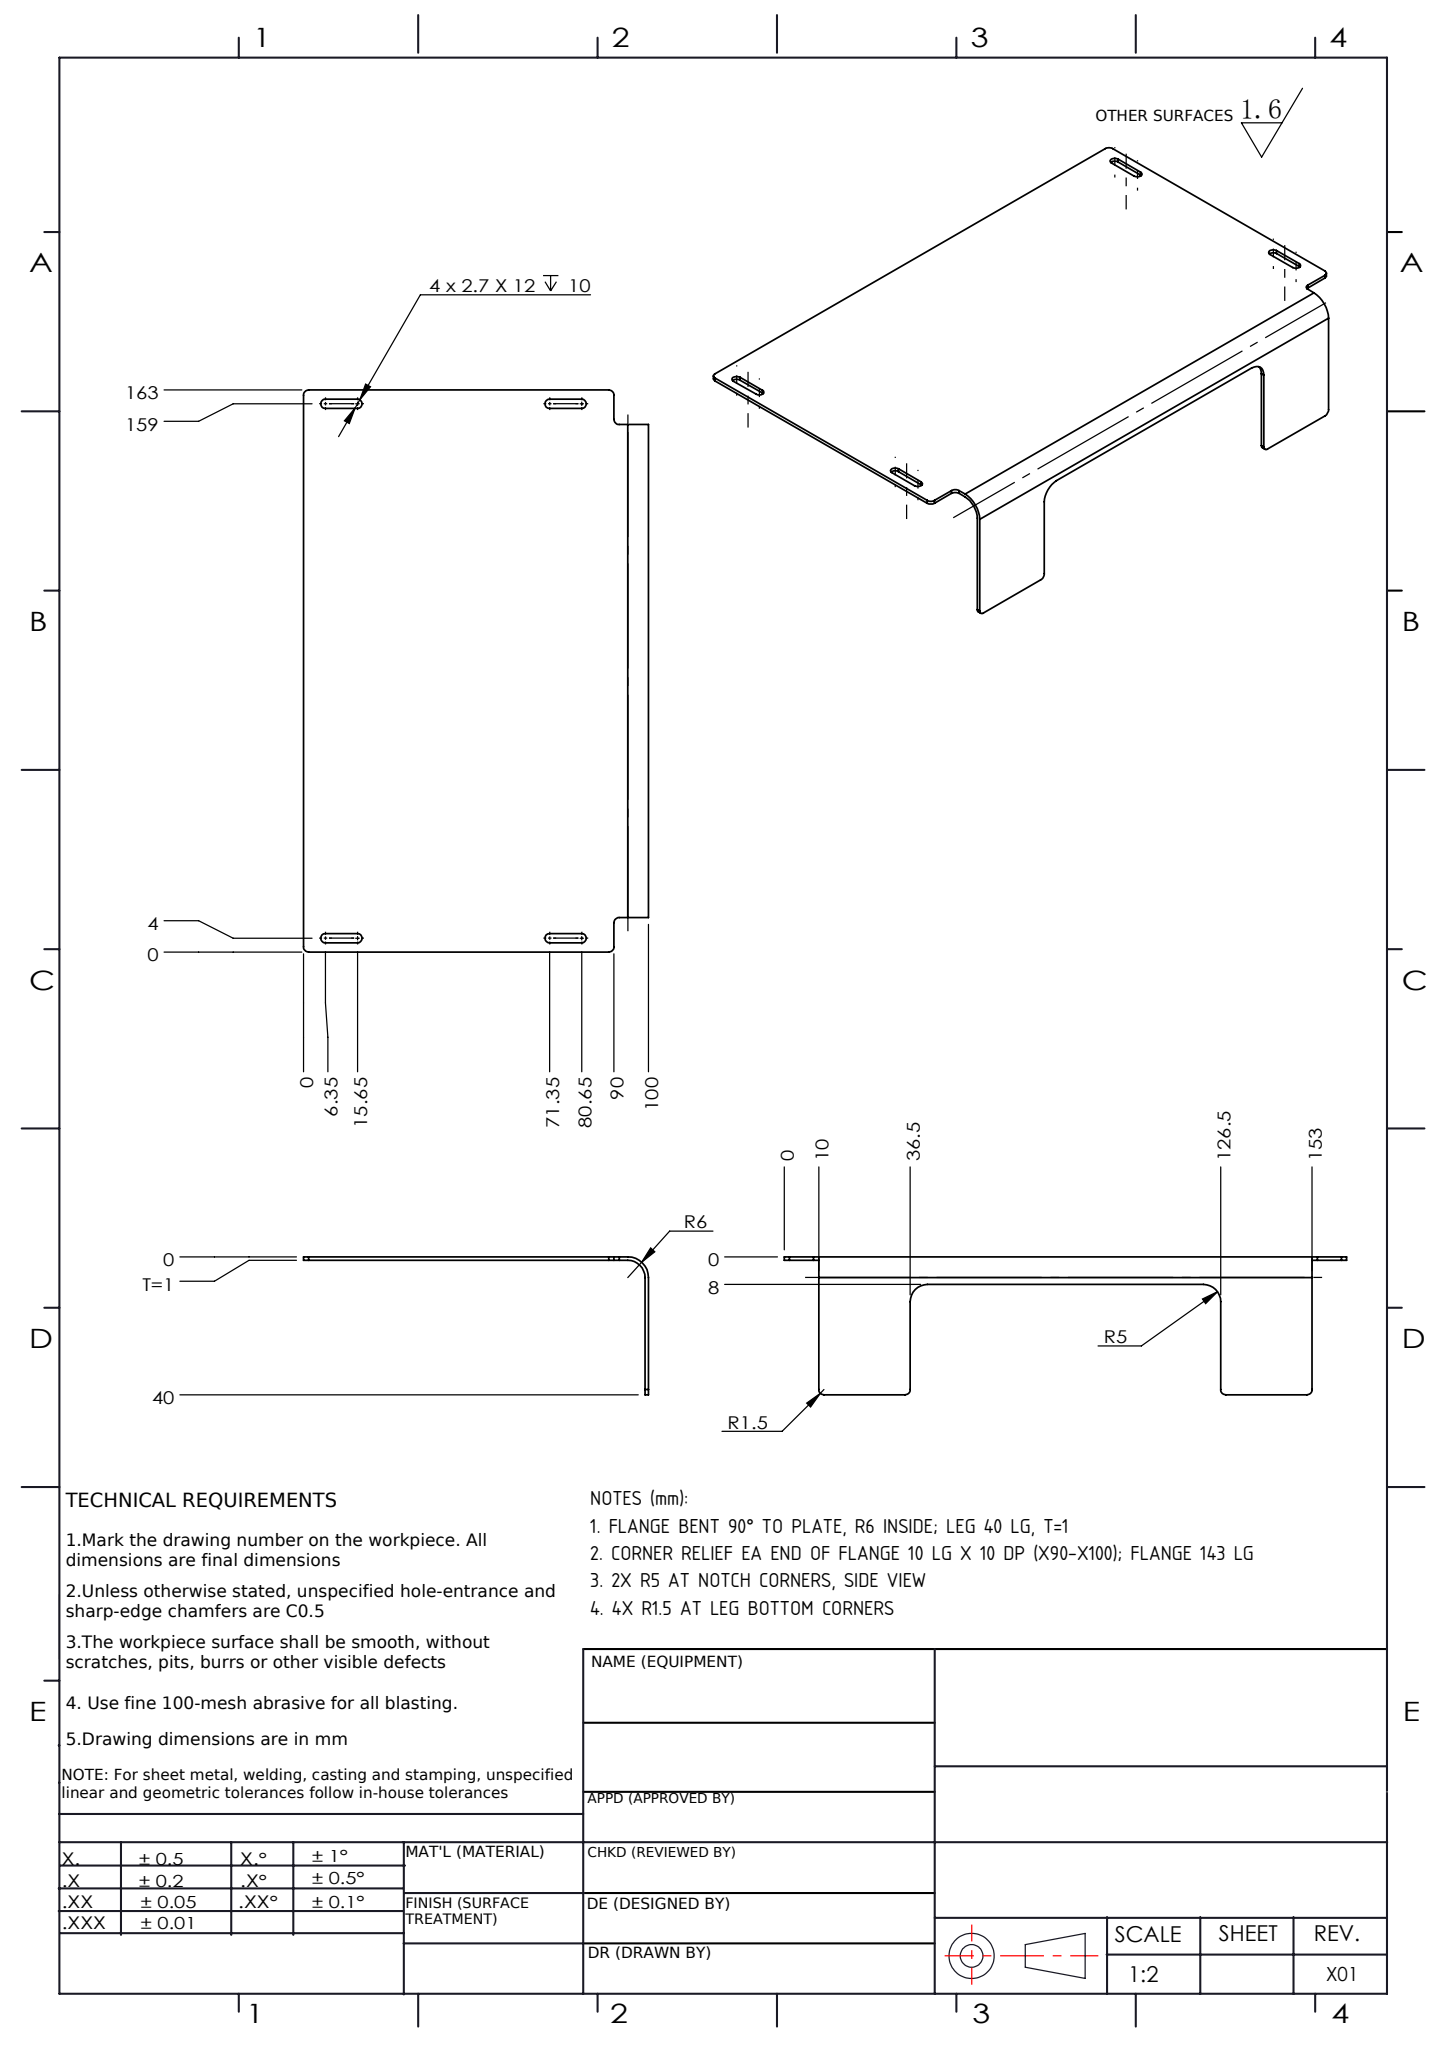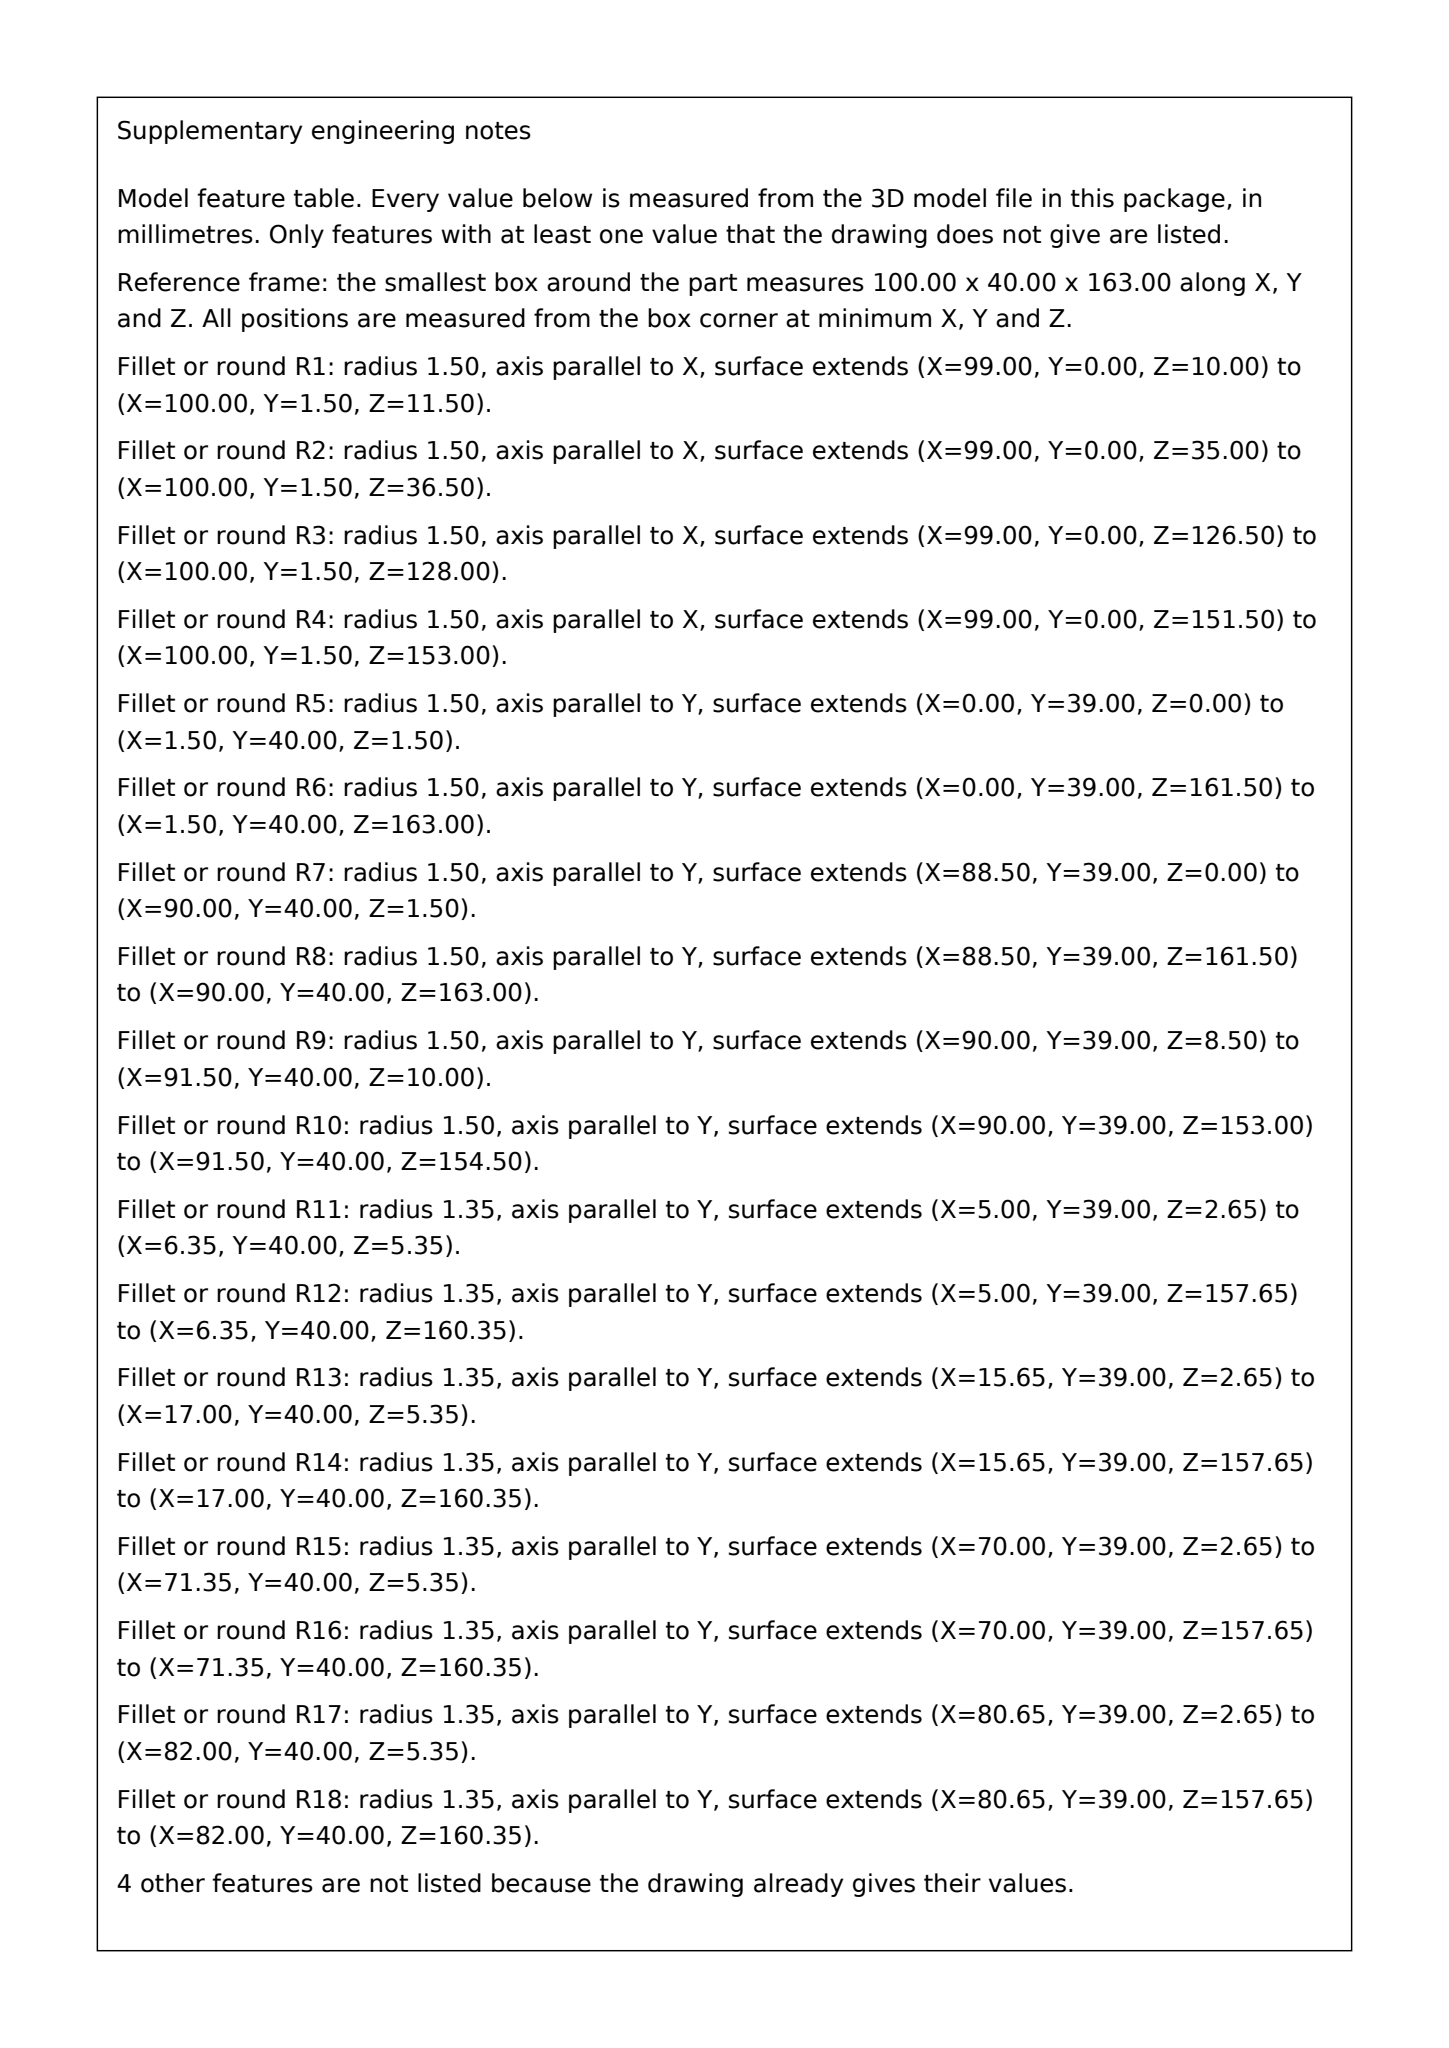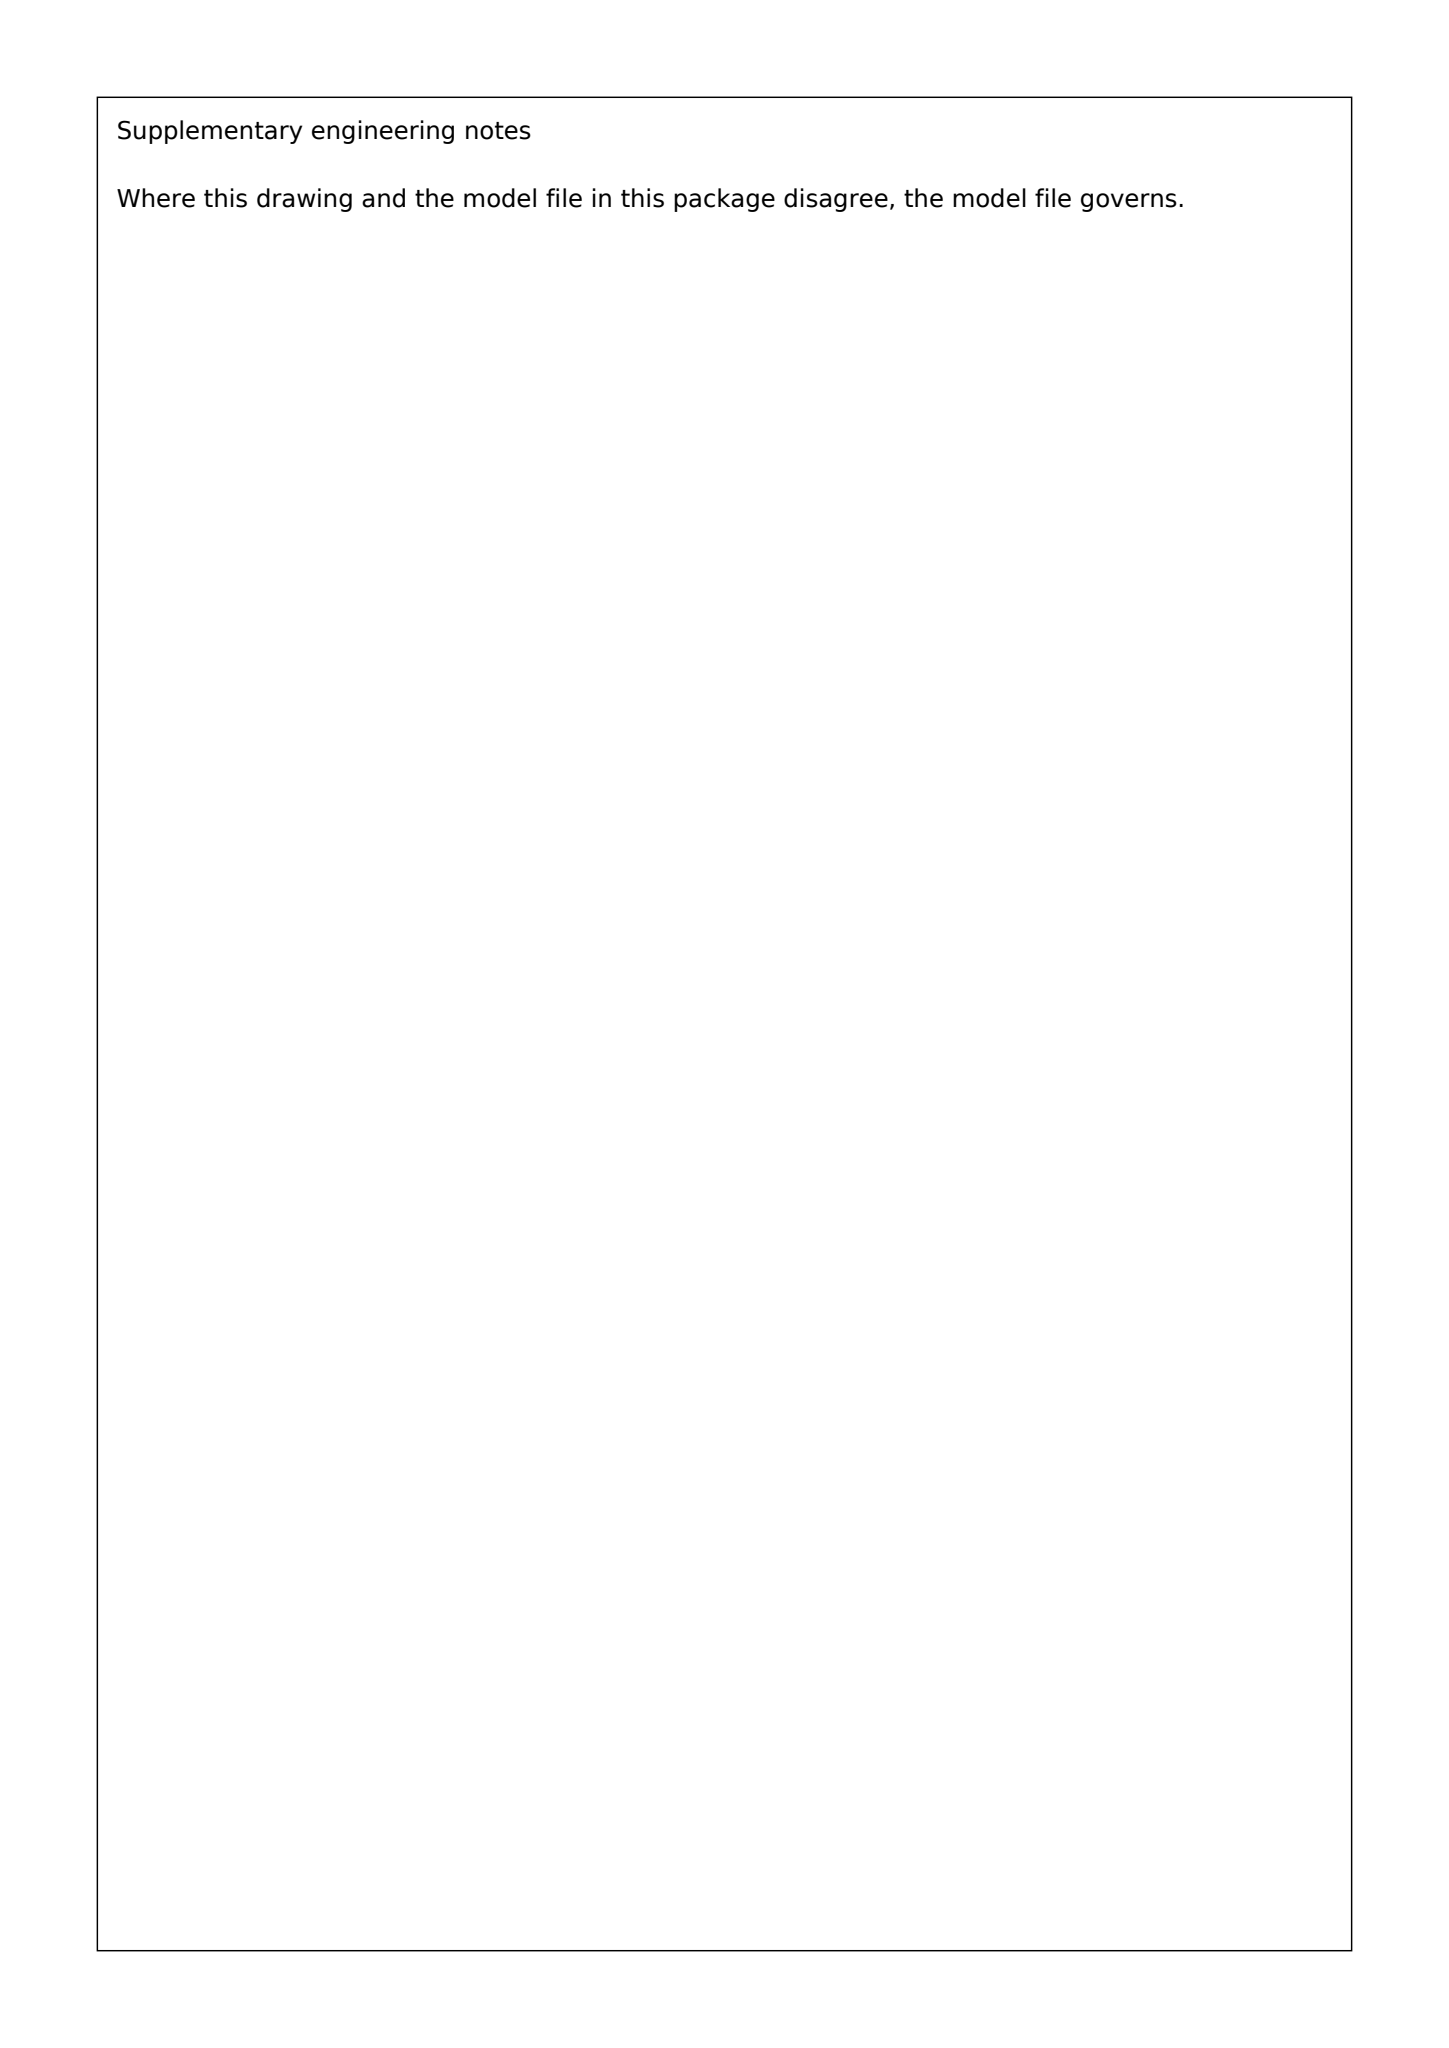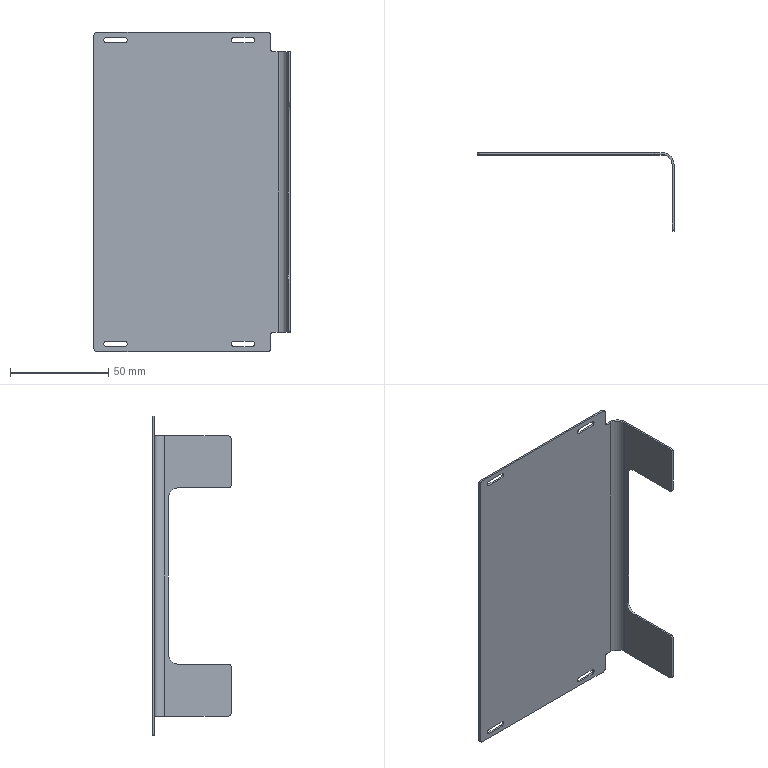Part | SolidWorks | mm | 1 solid | 46 faces | box 100 x 40 x 163 mm | volume 18344 mm3 | plane 24 | cylinder 22 | commonest cylinder face diameters 3 x10 2.7 x8 10 x3 12 x1
Drawing notes:
FLANGE BENT 90° TO PLATE, R6 INSIDE; LEG 40 LG, T=1 | from the solid: Flange faces perpendicular (90°) to plate; leg height 40, thickness 1
CORNER RELIEF EA END OF FLANGE 10 LG X 10 DP (X90-X100); FLANGE 143 LG | from the solid: z-planes 0/10/153/163; flange faces x=90..100 spanning z 10-153 (143 lg)
2X R5 AT NOTCH CORNERS, SIDE VIEW | from the solid: Ø10 cyl, axis x, at (y=27,z=41.5) and (y=27,z=121.5) => R5 x2
4X R1.5 AT LEG BOTTOM CORNERS | from the solid: Ø3 cyl, axis x, at y=1.5, z=11.5/35.0/128.0/151.5 => R1.5 x4